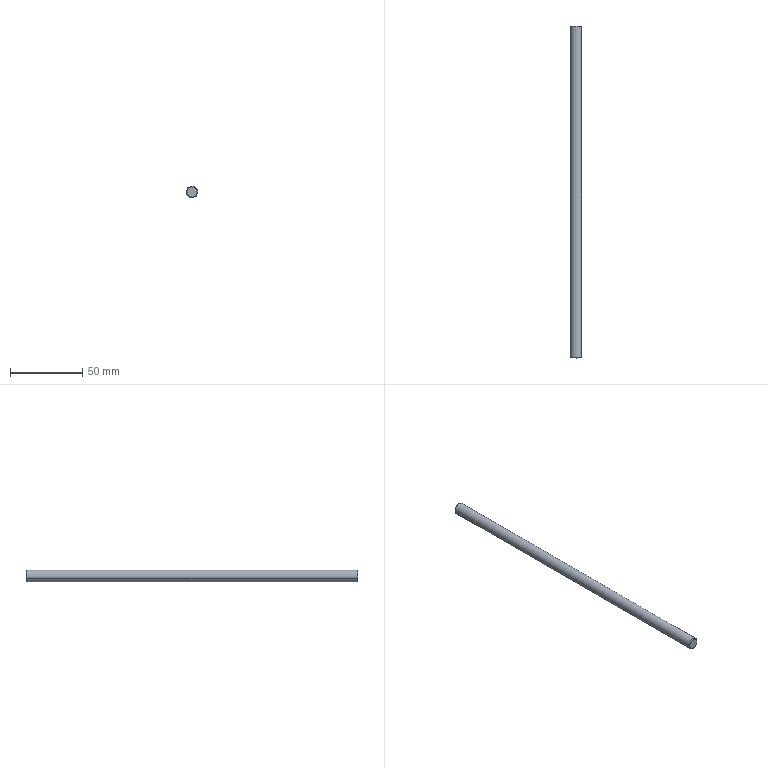Component | SolidWorks | SFJT8-230-M5-2 | 1 solid | 12 faces | box 8 x 230 x 8 mm | volume 11270 mm3 | cone 6 | cylinder 4 | plane 2 | commonest cylinder face diameters 5 x2 8 x2
build123d program:
from build123d import *

# Parameters (mm, degrees)
SKETCH1_R             = 4
EXTRUDE1_DEPTH        = 230
M5_TAPPED_HOLE1_D     = 5
M5_TAPPED_HOLE1_DEPTH = 14
M5_TAPPED_HOLE1_TIP   = 1.502
CHAMFER1_SIZE         = 0.5


with BuildPart() as part:
    # Sketch1 → Extrude1 (new body)
    with BuildSketch(Plane(origin=(0, 0, 0), x_dir=(1, 0, 0), z_dir=(0, 1, 0))):
        with Locations(Location((0, 0, 0), (0, 0, 270))):
            Circle(SKETCH1_R)
    extrude(amount=EXTRUDE1_DEPTH)

    # M5 Tapped Hole1
    with Locations(Plane.XZ):
        with Locations((0, 0)):
            Hole(M5_TAPPED_HOLE1_D / 2, depth=M5_TAPPED_HOLE1_DEPTH)
            with Locations((0, 0, -(M5_TAPPED_HOLE1_DEPTH + M5_TAPPED_HOLE1_TIP / 2))):  # 118° drill point
                Cone(0, M5_TAPPED_HOLE1_D / 2, M5_TAPPED_HOLE1_TIP, mode=Mode.SUBTRACT)

    # Chamfer1
    chamfer1_edges = [part.edges().sort_by_distance(p)[0] for p in [
        (0, 0, -4),
        (0, 230, -4),
    ]]
    chamfer(chamfer1_edges, length=CHAMFER1_SIZE)


solid = part.part

# Placed as in the assembly
solid = solid.moved(Location((-37.5, 195, -20), (180, 0, 0)))
STEP:
#1=COLOUR_RGB('',0.7922,0.8196,0.9333);
#2=FILL_AREA_STYLE_COLOUR('',#1);
#3=FILL_AREA_STYLE('',(#2));
#4=SURFACE_STYLE_FILL_AREA(#3);
#5=SURFACE_SIDE_STYLE('',(#4));
#6=SURFACE_STYLE_USAGE(.BOTH.,#5);
#7=PRESENTATION_STYLE_ASSIGNMENT((#6));
#8=CARTESIAN_POINT('',(-1.351,7.677,-0.7304));
#9=VERTEX_POINT('',#8);
#10=CARTESIAN_POINT('',(-1.602,7.677,-0.8444));
#11=VERTEX_POINT('',#10);
#12=CARTESIAN_POINT('',(-1.476,7.677,-0.7874));
#13=DIRECTION('',(-0.,1.,0.));
#14=DIRECTION('',(-0.9105,0.,-0.4136));
#15=AXIS2_PLACEMENT_3D('',#12,#13,#14);
#16=CIRCLE('',#15,0.1378);
#17=EDGE_CURVE('',#9,#11,#16,.T.);
#18=ORIENTED_EDGE('',*,*,#17,.F.);
#19=CARTESIAN_POINT('',(-1.333,7.657,-0.7223));
#20=VERTEX_POINT('',#19);
#21=CARTESIAN_POINT('',(-1.333,7.657,-0.7223));
#22=DIRECTION('',(0.6438,-0.7071,0.2924));
#23=VECTOR('',#22,39.37);
#24=LINE('',#21,#23);
#25=EDGE_CURVE('',#9,#20,#24,.T.);
#26=ORIENTED_EDGE('',*,*,#25,.T.);
#27=CARTESIAN_POINT('',(-1.62,7.657,-0.8525));
#28=VERTEX_POINT('',#27);
#29=CARTESIAN_POINT('',(-1.476,7.657,-0.7874));
#30=DIRECTION('',(0.,-1.,-0.));
#31=DIRECTION('',(-0.9105,0.,-0.4136));
#32=AXIS2_PLACEMENT_3D('',#29,#30,#31);
#33=CIRCLE('',#32,0.1575);
#34=EDGE_CURVE('',#28,#20,#33,.T.);
#35=ORIENTED_EDGE('',*,*,#34,.F.);
#36=CARTESIAN_POINT('',(-1.62,7.657,-0.8525));
#37=DIRECTION('',(-0.6438,-0.7071,-0.2924));
#38=VECTOR('',#37,39.37);
#39=LINE('',#36,#38);
#40=EDGE_CURVE('',#11,#28,#39,.T.);
#41=ORIENTED_EDGE('',*,*,#40,.F.);
#42=EDGE_LOOP('',(#18,#26,#35,#41));
#43=FACE_OUTER_BOUND('',#42,.T.);
#44=CARTESIAN_POINT('',(-1.476,7.657,-0.7874));
#45=DIRECTION('',(0.,-1.,-0.));
#46=DIRECTION('',(-0.9105,0.,-0.4136));
#47=AXIS2_PLACEMENT_3D('',#44,#45,#46);
#48=CONICAL_SURFACE('',#47,0.1575,0.7854);
#49=ADVANCED_FACE('',(#43),#48,.T.);
#50=CARTESIAN_POINT('',(-1.602,-1.378,-0.8444));
#51=VERTEX_POINT('',#50);
#52=CARTESIAN_POINT('',(-1.351,-1.378,-0.7304));
#53=VERTEX_POINT('',#52);
#54=CARTESIAN_POINT('',(-1.476,-1.378,-0.7874));
#55=DIRECTION('',(0.,-1.,-0.));
#56=DIRECTION('',(-0.9105,0.,-0.4136));
#57=AXIS2_PLACEMENT_3D('',#54,#55,#56);
#58=CIRCLE('',#57,0.1378);
#59=EDGE_CURVE('',#51,#53,#58,.T.);
#60=ORIENTED_EDGE('',*,*,#59,.F.);
#61=CARTESIAN_POINT('',(-1.62,-1.358,-0.8525));
#62=VERTEX_POINT('',#61);
#63=CARTESIAN_POINT('',(-1.602,-1.378,-0.8444));
#64=DIRECTION('',(-0.6438,0.7071,-0.2924));
#65=VECTOR('',#64,39.37);
#66=LINE('',#63,#65);
#67=EDGE_CURVE('',#51,#62,#66,.T.);
#68=ORIENTED_EDGE('',*,*,#67,.T.);
#69=CARTESIAN_POINT('',(-1.333,-1.358,-0.7223));
#70=VERTEX_POINT('',#69);
#71=CARTESIAN_POINT('',(-1.476,-1.358,-0.7874));
#72=DIRECTION('',(-0.,1.,0.));
#73=DIRECTION('',(-0.9105,0.,-0.4136));
#74=AXIS2_PLACEMENT_3D('',#71,#72,#73);
#75=CIRCLE('',#74,0.1575);
#76=EDGE_CURVE('',#70,#62,#75,.T.);
#77=ORIENTED_EDGE('',*,*,#76,.F.);
#78=CARTESIAN_POINT('',(-1.351,-1.378,-0.7304));
#79=DIRECTION('',(0.6438,0.7071,0.2924));
#80=VECTOR('',#79,39.37);
#81=LINE('',#78,#80);
#82=EDGE_CURVE('',#53,#70,#81,.T.);
#83=ORIENTED_EDGE('',*,*,#82,.F.);
#84=EDGE_LOOP('',(#60,#68,#77,#83));
#85=FACE_OUTER_BOUND('',#84,.T.);
#86=CARTESIAN_POINT('',(-1.476,-1.378,-0.7874));
#87=DIRECTION('',(-0.,1.,0.));
#88=DIRECTION('',(0.9105,0.,0.4136));
#89=AXIS2_PLACEMENT_3D('',#86,#87,#88);
#90=CONICAL_SURFACE('',#89,0.1378,0.7854);
#91=ADVANCED_FACE('',(#85),#90,.T.);
#92=CARTESIAN_POINT('',(-1.476,7.067,-0.7874));
#93=VERTEX_POINT('',#92);
#94=CARTESIAN_POINT('',(-1.387,7.126,-0.7467));
#95=VERTEX_POINT('',#94);
#96=CARTESIAN_POINT('',(-1.387,7.126,-0.7467));
#97=DIRECTION('',(0.7804,0.515,0.3545));
#98=VECTOR('',#97,39.37);
#99=LINE('',#96,#98);
#100=EDGE_CURVE('',#93,#95,#99,.T.);
#101=ORIENTED_EDGE('',*,*,#100,.F.);
#102=CARTESIAN_POINT('',(-1.566,7.126,-0.8281));
#103=VERTEX_POINT('',#102);
#104=CARTESIAN_POINT('',(-1.566,7.126,-0.8281));
#105=DIRECTION('',(-0.7804,0.515,-0.3545));
#106=VECTOR('',#105,39.37);
#107=LINE('',#104,#106);
#108=EDGE_CURVE('',#93,#103,#107,.T.);
#109=ORIENTED_EDGE('',*,*,#108,.T.);
#110=CARTESIAN_POINT('',(-1.476,7.126,-0.7874));
#111=DIRECTION('',(-0.,1.,0.));
#112=DIRECTION('',(0.9105,0.,0.4136));
#113=AXIS2_PLACEMENT_3D('',#110,#111,#112);
#114=CIRCLE('',#113,0.09843);
#115=EDGE_CURVE('',#103,#95,#114,.T.);
#116=ORIENTED_EDGE('',*,*,#115,.T.);
#117=EDGE_LOOP('',(#101,#109,#116));
#118=FACE_OUTER_BOUND('',#117,.T.);
#119=CARTESIAN_POINT('',(-1.476,7.126,-0.7874));
#120=DIRECTION('',(-0.,1.,0.));
#121=DIRECTION('',(0.9105,0.,0.4136));
#122=AXIS2_PLACEMENT_3D('',#119,#120,#121);
#123=CONICAL_SURFACE('',#122,0.09843,1.03);
#124=ADVANCED_FACE('',(#118),#123,.F.);
#125=ORIENTED_EDGE('',*,*,#115,.F.);
#126=CARTESIAN_POINT('',(-1.566,7.677,-0.8281));
#127=VERTEX_POINT('',#126);
#128=CARTESIAN_POINT('',(-1.566,7.677,-0.8281));
#129=DIRECTION('',(-0.,1.,0.));
#130=VECTOR('',#129,39.37);
#131=LINE('',#128,#130);
#132=EDGE_CURVE('',#103,#127,#131,.T.);
#133=ORIENTED_EDGE('',*,*,#132,.T.);
#134=CARTESIAN_POINT('',(-1.387,7.677,-0.7467));
#135=VERTEX_POINT('',#134);
#136=CARTESIAN_POINT('',(-1.476,7.677,-0.7874));
#137=DIRECTION('',(-0.,1.,0.));
#138=DIRECTION('',(0.9105,0.,0.4136));
#139=AXIS2_PLACEMENT_3D('',#136,#137,#138);
#140=CIRCLE('',#139,0.09843);
#141=EDGE_CURVE('',#127,#135,#140,.T.);
#142=ORIENTED_EDGE('',*,*,#141,.T.);
#143=CARTESIAN_POINT('',(-1.387,7.677,-0.7467));
#144=DIRECTION('',(-0.,1.,0.));
#145=VECTOR('',#144,39.37);
#146=LINE('',#143,#145);
#147=EDGE_CURVE('',#95,#135,#146,.T.);
#148=ORIENTED_EDGE('',*,*,#147,.F.);
#149=EDGE_LOOP('',(#125,#133,#142,#148));
#150=FACE_OUTER_BOUND('',#149,.T.);
#151=CARTESIAN_POINT('',(-1.476,7.677,-0.7874));
#152=DIRECTION('',(-0.,1.,0.));
#153=DIRECTION('',(0.9105,0.,0.4136));
#154=AXIS2_PLACEMENT_3D('',#151,#152,#153);
#155=CYLINDRICAL_SURFACE('',#154,0.09843);
#156=ADVANCED_FACE('',(#150),#155,.F.);
#157=ORIENTED_EDGE('',*,*,#76,.T.);
#158=CARTESIAN_POINT('',(-1.62,-1.378,-0.8525));
#159=DIRECTION('',(-0.,1.,0.));
#160=VECTOR('',#159,39.37);
#161=LINE('',#158,#160);
#162=EDGE_CURVE('',#62,#28,#161,.T.);
#163=ORIENTED_EDGE('',*,*,#162,.T.);
#164=ORIENTED_EDGE('',*,*,#34,.T.);
#165=CARTESIAN_POINT('',(-1.333,-1.378,-0.7223));
#166=DIRECTION('',(-0.,1.,0.));
#167=VECTOR('',#166,39.37);
#168=LINE('',#165,#167);
#169=EDGE_CURVE('',#70,#20,#168,.T.);
#170=ORIENTED_EDGE('',*,*,#169,.F.);
#171=EDGE_LOOP('',(#157,#163,#164,#170));
#172=FACE_OUTER_BOUND('',#171,.T.);
#173=CARTESIAN_POINT('',(-1.476,-1.378,-0.7874));
#174=DIRECTION('',(-0.,1.,0.));
#175=DIRECTION('',(0.9105,0.,0.4136));
#176=AXIS2_PLACEMENT_3D('',#173,#174,#175);
#177=CYLINDRICAL_SURFACE('',#176,0.1575);
#178=ADVANCED_FACE('',(#172),#177,.T.);
#179=ORIENTED_EDGE('',*,*,#162,.F.);
#180=CARTESIAN_POINT('',(-1.476,-1.358,-0.7874));
#181=DIRECTION('',(-0.,1.,0.));
#182=DIRECTION('',(-0.9105,0.,-0.4136));
#183=AXIS2_PLACEMENT_3D('',#180,#181,#182);
#184=CIRCLE('',#183,0.1575);
#185=EDGE_CURVE('',#62,#70,#184,.T.);
#186=ORIENTED_EDGE('',*,*,#185,.T.);
#187=ORIENTED_EDGE('',*,*,#169,.T.);
#188=CARTESIAN_POINT('',(-1.476,7.657,-0.7874));
#189=DIRECTION('',(0.,-1.,-0.));
#190=DIRECTION('',(-0.9105,0.,-0.4136));
#191=AXIS2_PLACEMENT_3D('',#188,#189,#190);
#192=CIRCLE('',#191,0.1575);
#193=EDGE_CURVE('',#20,#28,#192,.T.);
#194=ORIENTED_EDGE('',*,*,#193,.T.);
#195=EDGE_LOOP('',(#179,#186,#187,#194));
#196=FACE_OUTER_BOUND('',#195,.T.);
#197=CARTESIAN_POINT('',(-1.476,-1.378,-0.7874));
#198=DIRECTION('',(-0.,1.,0.));
#199=DIRECTION('',(0.9105,0.,0.4136));
#200=AXIS2_PLACEMENT_3D('',#197,#198,#199);
#201=CYLINDRICAL_SURFACE('',#200,0.1575);
#202=ADVANCED_FACE('',(#196),#201,.T.);
#203=CARTESIAN_POINT('',(-1.476,-1.378,-0.7874));
#204=DIRECTION('',(0.,-1.,-0.));
#205=DIRECTION('',(-0.9105,0.,-0.4136));
#206=AXIS2_PLACEMENT_3D('',#203,#204,#205);
#207=CIRCLE('',#206,0.1378);
#208=EDGE_CURVE('',#53,#51,#207,.T.);
#209=ORIENTED_EDGE('',*,*,#208,.T.);
#210=ORIENTED_EDGE('',*,*,#59,.T.);
#211=EDGE_LOOP('',(#209,#210));
#212=FACE_OUTER_BOUND('',#211,.T.);
#213=CARTESIAN_POINT('',(-1.476,-1.378,-0.7874));
#214=DIRECTION('',(0.,-1.,-0.));
#215=DIRECTION('',(-0.9105,0.,-0.4136));
#216=AXIS2_PLACEMENT_3D('',#213,#214,#215);
#217=PLANE('',#216);
#218=ADVANCED_FACE('',(#212),#217,.T.);
#219=CARTESIAN_POINT('',(-1.476,7.677,-0.7874));
#220=DIRECTION('',(-0.,1.,0.));
#221=DIRECTION('',(-0.9105,0.,-0.4136));
#222=AXIS2_PLACEMENT_3D('',#219,#220,#221);
#223=CIRCLE('',#222,0.1378);
#224=EDGE_CURVE('',#11,#9,#223,.T.);
#225=ORIENTED_EDGE('',*,*,#224,.T.);
#226=ORIENTED_EDGE('',*,*,#17,.T.);
#227=EDGE_LOOP('',(#225,#226));
#228=FACE_OUTER_BOUND('',#227,.T.);
#229=CARTESIAN_POINT('',(-1.476,7.677,-0.7874));
#230=DIRECTION('',(-0.,1.,0.));
#231=DIRECTION('',(0.9105,0.,0.4136));
#232=AXIS2_PLACEMENT_3D('',#229,#230,#231);
#233=CIRCLE('',#232,0.09843);
#234=EDGE_CURVE('',#135,#127,#233,.T.);
#235=ORIENTED_EDGE('',*,*,#234,.F.);
#236=ORIENTED_EDGE('',*,*,#141,.F.);
#237=EDGE_LOOP('',(#235,#236));
#238=FACE_BOUND('',#237,.T.);
#239=CARTESIAN_POINT('',(-1.476,7.677,-0.7874));
#240=DIRECTION('',(0.,-1.,-0.));
#241=DIRECTION('',(-0.9105,0.,-0.4136));
#242=AXIS2_PLACEMENT_3D('',#239,#240,#241);
#243=PLANE('',#242);
#244=ADVANCED_FACE('',(#228,#238),#243,.F.);
#245=ORIENTED_EDGE('',*,*,#132,.F.);
#246=CARTESIAN_POINT('',(-1.476,7.126,-0.7874));
#247=DIRECTION('',(-0.,1.,0.));
#248=DIRECTION('',(0.9105,0.,0.4136));
#249=AXIS2_PLACEMENT_3D('',#246,#247,#248);
#250=CIRCLE('',#249,0.09843);
#251=EDGE_CURVE('',#95,#103,#250,.T.);
#252=ORIENTED_EDGE('',*,*,#251,.F.);
#253=ORIENTED_EDGE('',*,*,#147,.T.);
#254=ORIENTED_EDGE('',*,*,#234,.T.);
#255=EDGE_LOOP('',(#245,#252,#253,#254));
#256=FACE_OUTER_BOUND('',#255,.T.);
#257=CARTESIAN_POINT('',(-1.476,7.677,-0.7874));
#258=DIRECTION('',(-0.,1.,0.));
#259=DIRECTION('',(0.9105,0.,0.4136));
#260=AXIS2_PLACEMENT_3D('',#257,#258,#259);
#261=CYLINDRICAL_SURFACE('',#260,0.09843);
#262=ADVANCED_FACE('',(#256),#261,.F.);
#263=ORIENTED_EDGE('',*,*,#108,.F.);
#264=ORIENTED_EDGE('',*,*,#100,.T.);
#265=ORIENTED_EDGE('',*,*,#251,.T.);
#266=EDGE_LOOP('',(#263,#264,#265));
#267=FACE_OUTER_BOUND('',#266,.T.);
#268=CARTESIAN_POINT('',(-1.476,7.126,-0.7874));
#269=DIRECTION('',(-0.,1.,0.));
#270=DIRECTION('',(0.9105,0.,0.4136));
#271=AXIS2_PLACEMENT_3D('',#268,#269,#270);
#272=CONICAL_SURFACE('',#271,0.09843,1.03);
#273=ADVANCED_FACE('',(#267),#272,.F.);
#274=ORIENTED_EDGE('',*,*,#67,.F.);
#275=ORIENTED_EDGE('',*,*,#208,.F.);
#276=ORIENTED_EDGE('',*,*,#82,.T.);
#277=ORIENTED_EDGE('',*,*,#185,.F.);
#278=EDGE_LOOP('',(#274,#275,#276,#277));
#279=FACE_OUTER_BOUND('',#278,.T.);
#280=CARTESIAN_POINT('',(-1.476,-1.378,-0.7874));
#281=DIRECTION('',(-0.,1.,0.));
#282=DIRECTION('',(0.9105,0.,0.4136));
#283=AXIS2_PLACEMENT_3D('',#280,#281,#282);
#284=CONICAL_SURFACE('',#283,0.1378,0.7854);
#285=ADVANCED_FACE('',(#279),#284,.T.);
#286=ORIENTED_EDGE('',*,*,#25,.F.);
#287=ORIENTED_EDGE('',*,*,#224,.F.);
#288=ORIENTED_EDGE('',*,*,#40,.T.);
#289=ORIENTED_EDGE('',*,*,#193,.F.);
#290=EDGE_LOOP('',(#286,#287,#288,#289));
#291=FACE_OUTER_BOUND('',#290,.T.);
#292=CARTESIAN_POINT('',(-1.476,7.657,-0.7874));
#293=DIRECTION('',(0.,-1.,-0.));
#294=DIRECTION('',(-0.9105,0.,-0.4136));
#295=AXIS2_PLACEMENT_3D('',#292,#293,#294);
#296=CONICAL_SURFACE('',#295,0.1575,0.7854);
#297=ADVANCED_FACE('',(#291),#296,.T.);
#298=CLOSED_SHELL('',(#49,#91,#124,#156,#178,#202,#218,#244,#262,#273,#285,#297));
#299=MANIFOLD_SOLID_BREP('',#298);
#300=STYLED_ITEM('',(#7),#299);
#301=PRESENTATION_LAYER_ASSIGNMENT('','',(#300));
#302=(LENGTH_UNIT()NAMED_UNIT(*)SI_UNIT($,.METRE.));
#303=LENGTH_MEASURE_WITH_UNIT(LENGTH_MEASURE(0.0254),#302);
#304=DIMENSIONAL_EXPONENTS(1.,0.,0.,0.,0.,0.,0.);
#305=(CONVERSION_BASED_UNIT('',#303)LENGTH_UNIT()NAMED_UNIT(#304));
#306=UNCERTAINTY_MEASURE_WITH_UNIT(LENGTH_MEASURE(0.00001),#305,'','');
#307=(NAMED_UNIT(*)PLANE_ANGLE_UNIT()SI_UNIT($,.RADIAN.));
#308=(NAMED_UNIT(*)SI_UNIT($,.STERADIAN.)SOLID_ANGLE_UNIT());
#309=(GEOMETRIC_REPRESENTATION_CONTEXT(3)GLOBAL_UNCERTAINTY_ASSIGNED_CONTEXT((#306))GLOBAL_UNIT_ASSIGNED_CONTEXT((#305,#307,#308))REPRESENTATION_CONTEXT('',''));
#310=MECHANICAL_DESIGN_GEOMETRIC_PRESENTATION_REPRESENTATION('',(#300),#309);
#311=CARTESIAN_POINT('',(0.,0.,0.));
#312=DIRECTION('',(0.,0.,1.));
#313=DIRECTION('',(1.,0.,0.));
#314=AXIS2_PLACEMENT_3D('',#311,#312,#313);
#315=(LENGTH_UNIT()NAMED_UNIT(*)SI_UNIT($,.METRE.));
#316=LENGTH_MEASURE_WITH_UNIT(LENGTH_MEASURE(0.0254),#315);
#317=DIMENSIONAL_EXPONENTS(1.,0.,0.,0.,0.,0.,0.);
#318=(CONVERSION_BASED_UNIT('',#316)LENGTH_UNIT()NAMED_UNIT(#317));
#319=UNCERTAINTY_MEASURE_WITH_UNIT(LENGTH_MEASURE(0.00001),#318,'','');
#320=(NAMED_UNIT(*)PLANE_ANGLE_UNIT()SI_UNIT($,.RADIAN.));
#321=(NAMED_UNIT(*)SI_UNIT($,.STERADIAN.)SOLID_ANGLE_UNIT());
#322=(GEOMETRIC_REPRESENTATION_CONTEXT(3)GLOBAL_UNCERTAINTY_ASSIGNED_CONTEXT((#319))GLOBAL_UNIT_ASSIGNED_CONTEXT((#318,#320,#321))REPRESENTATION_CONTEXT('',''));
#323=ADVANCED_BREP_SHAPE_REPRESENTATION('',(#299,#314),#322);